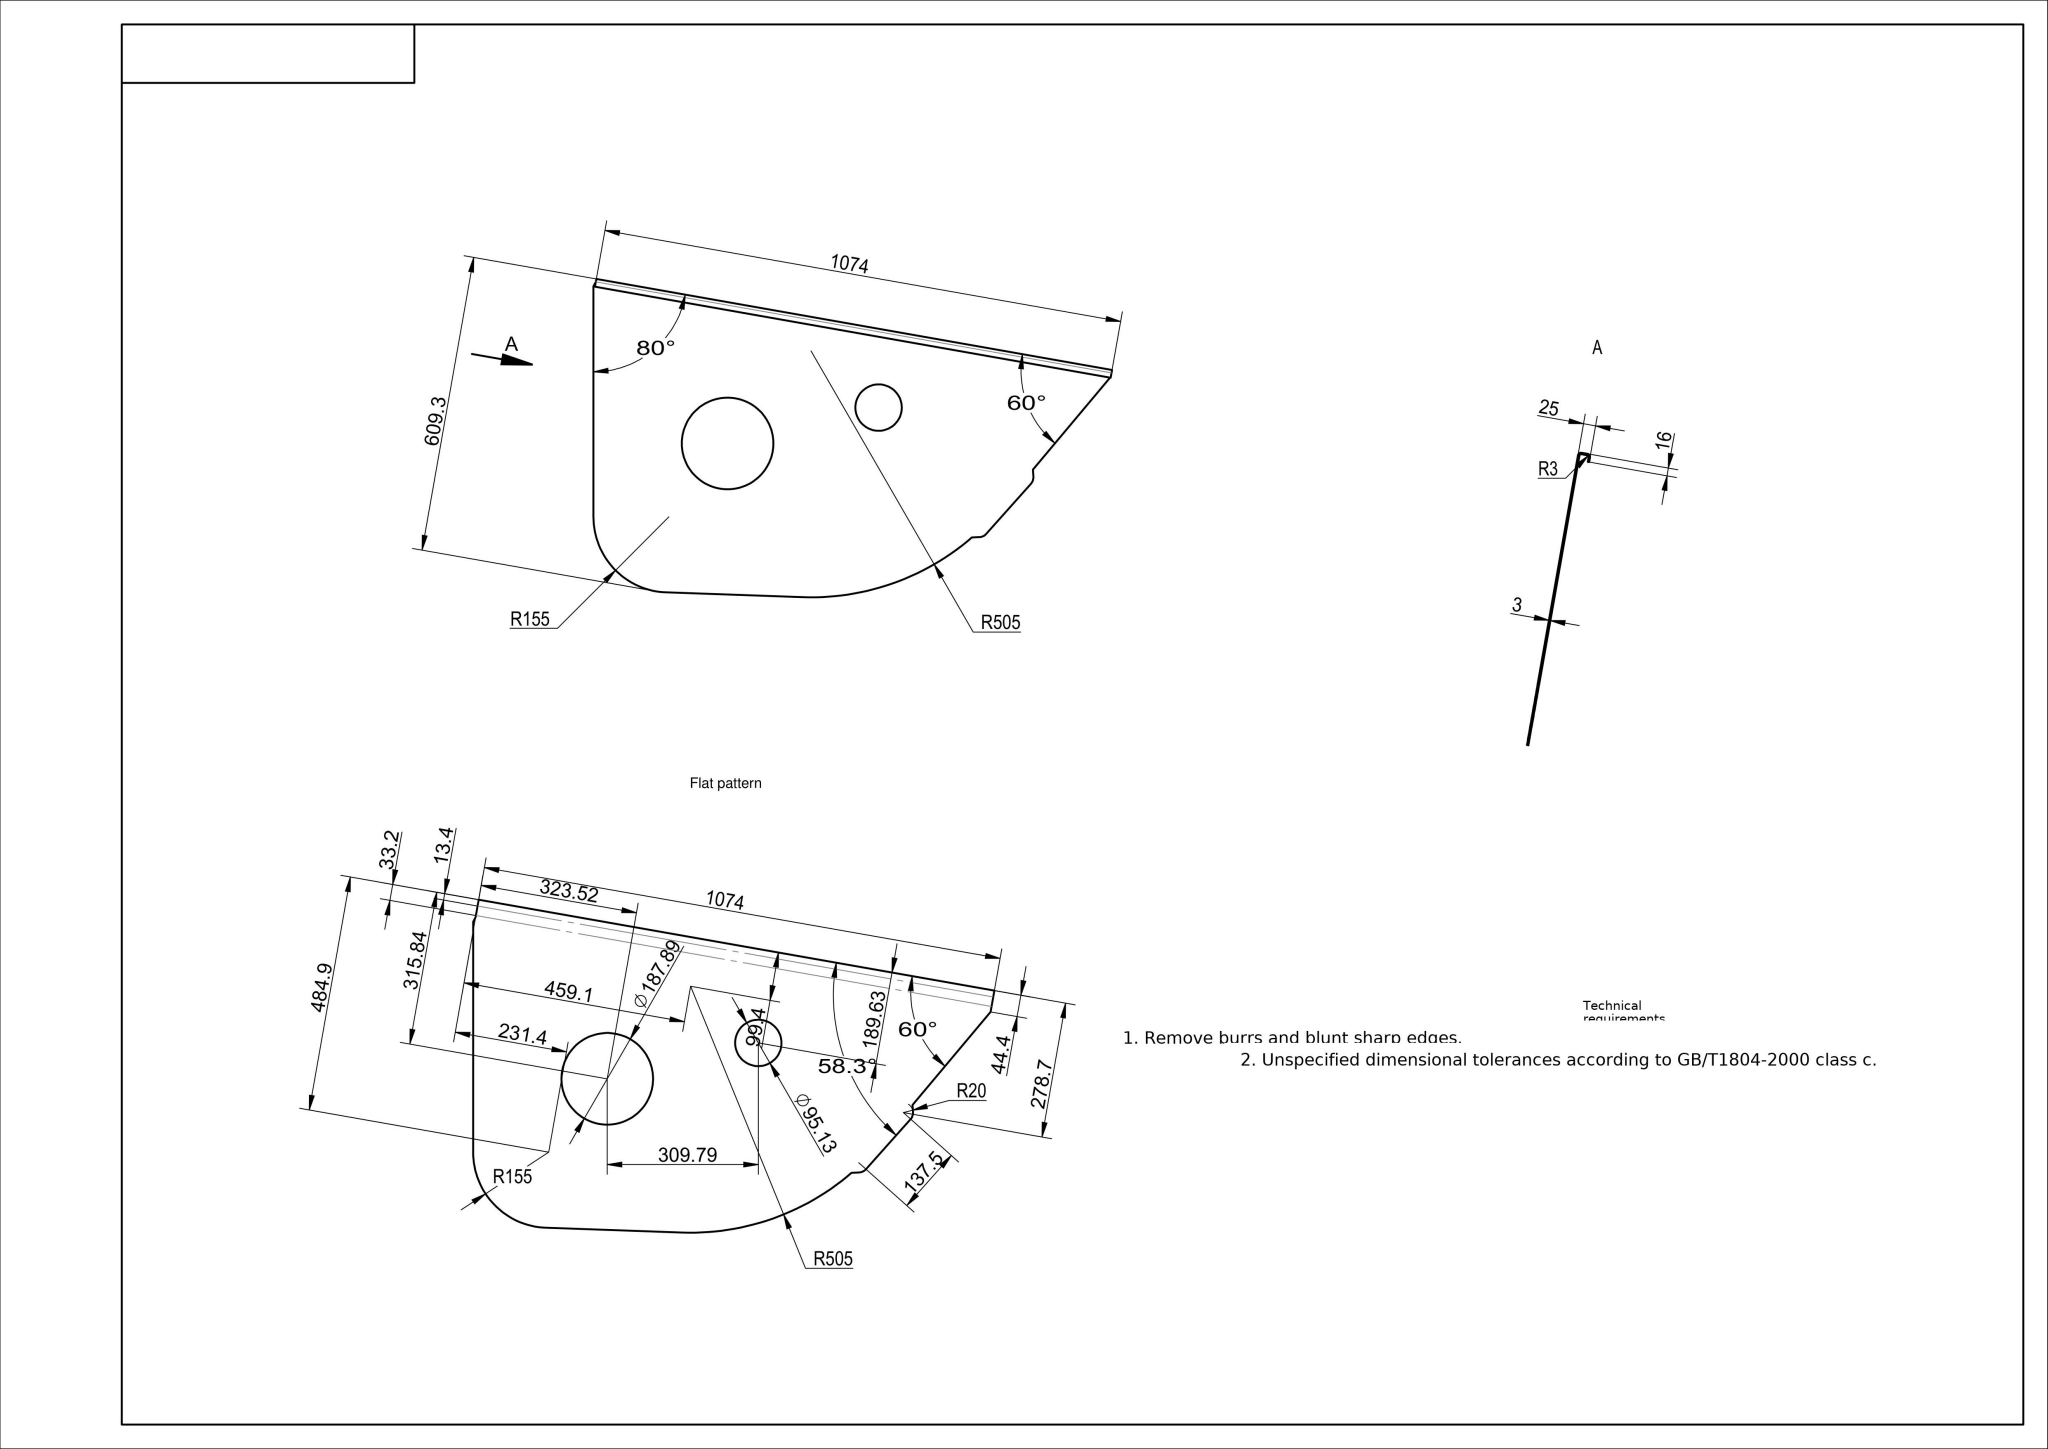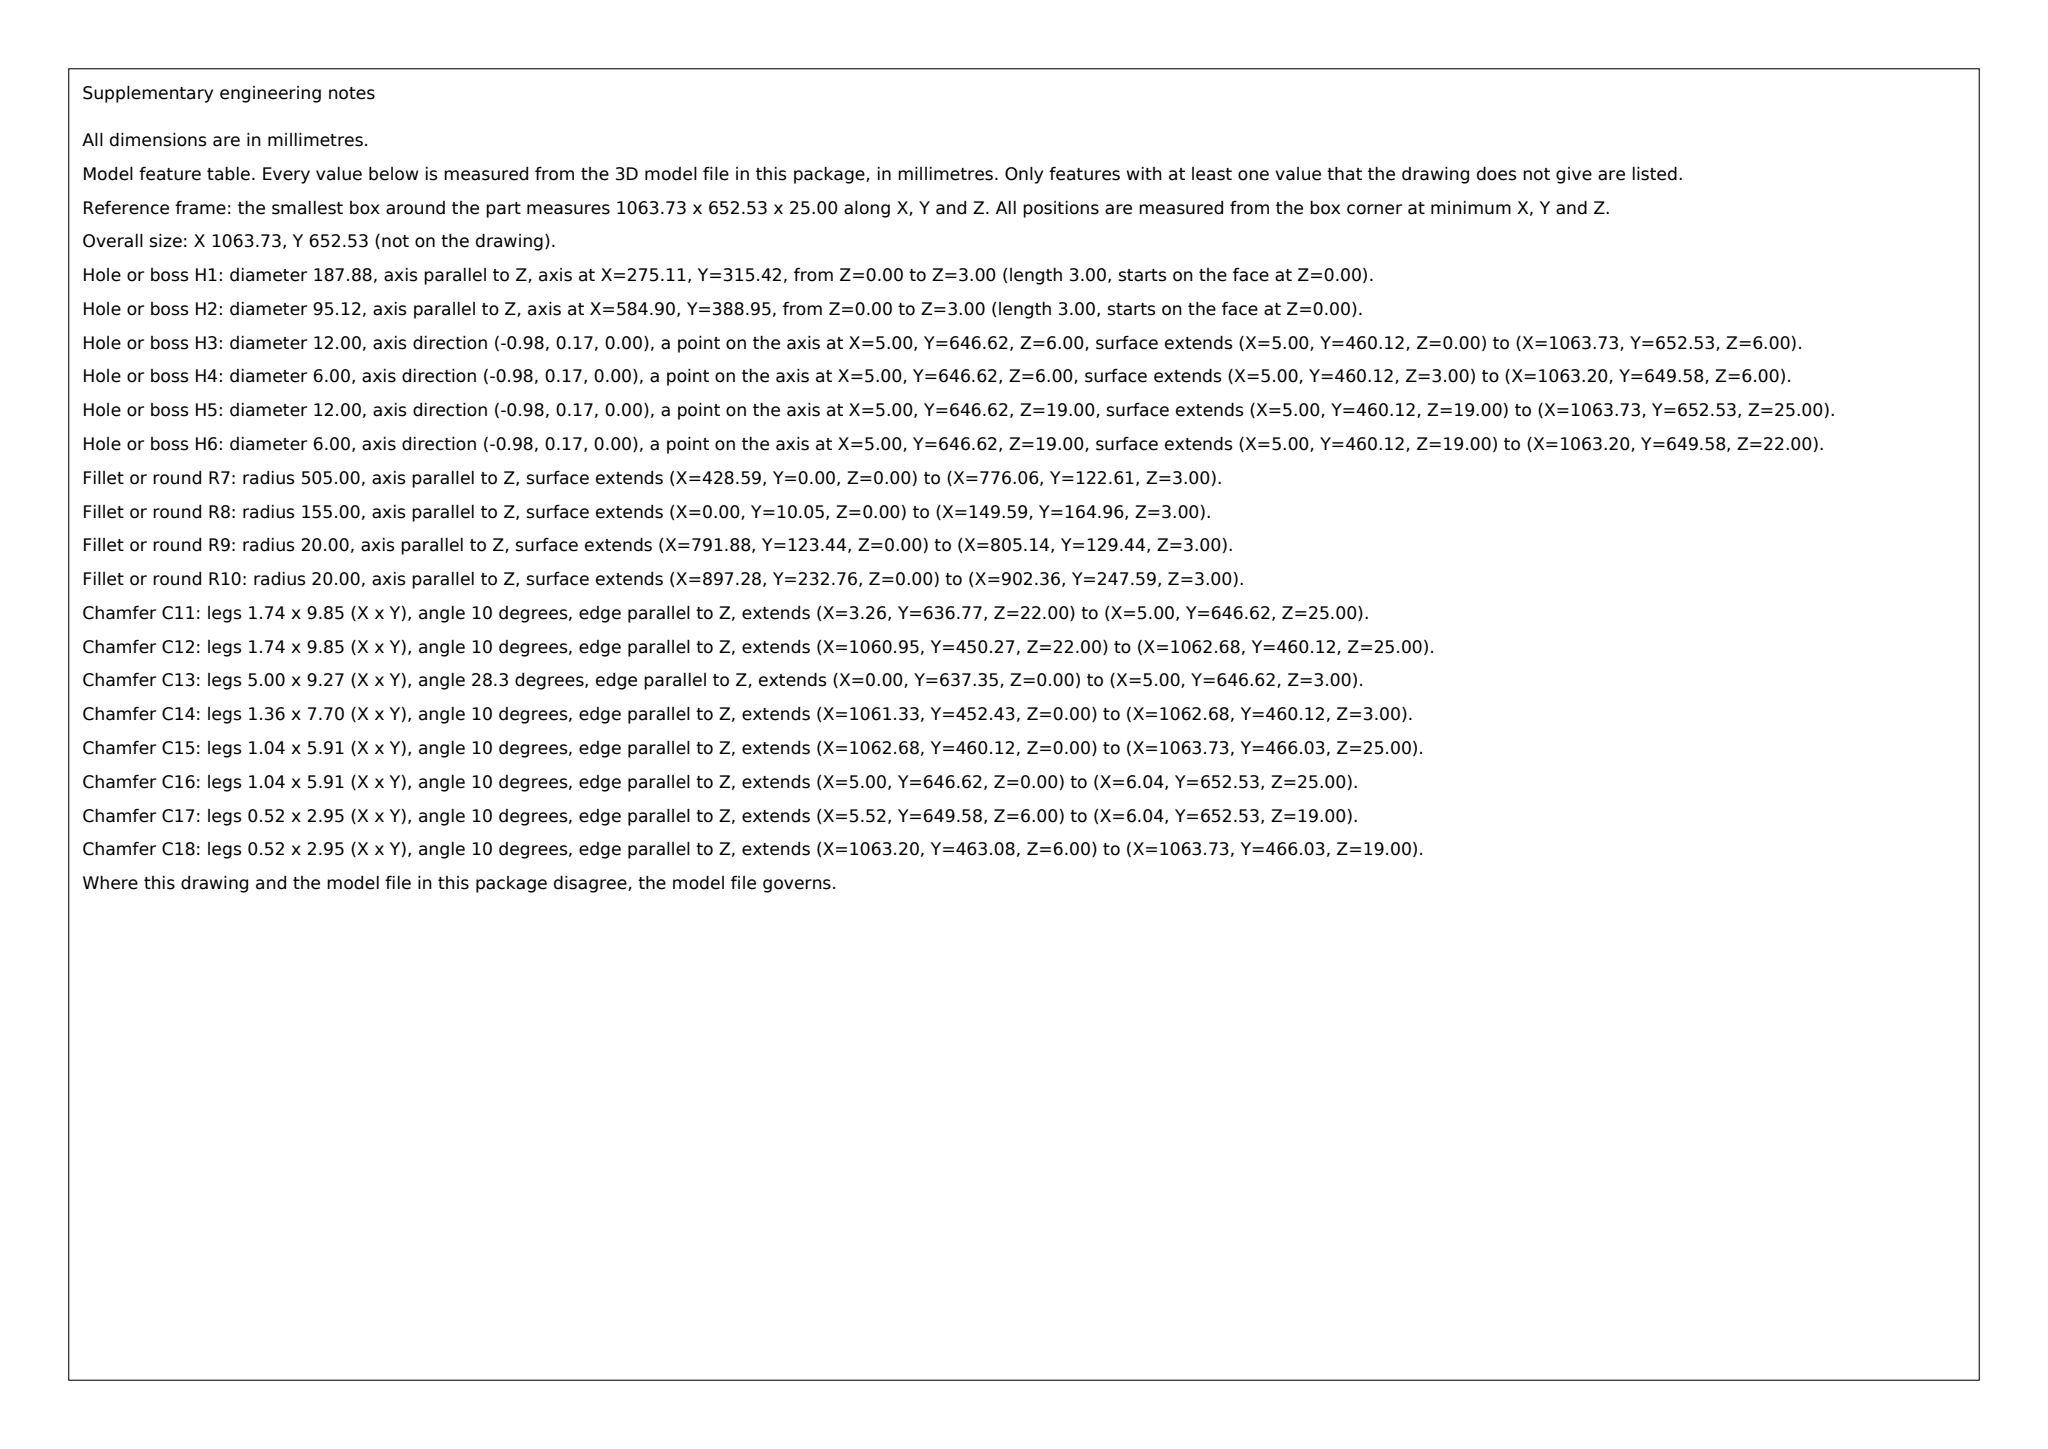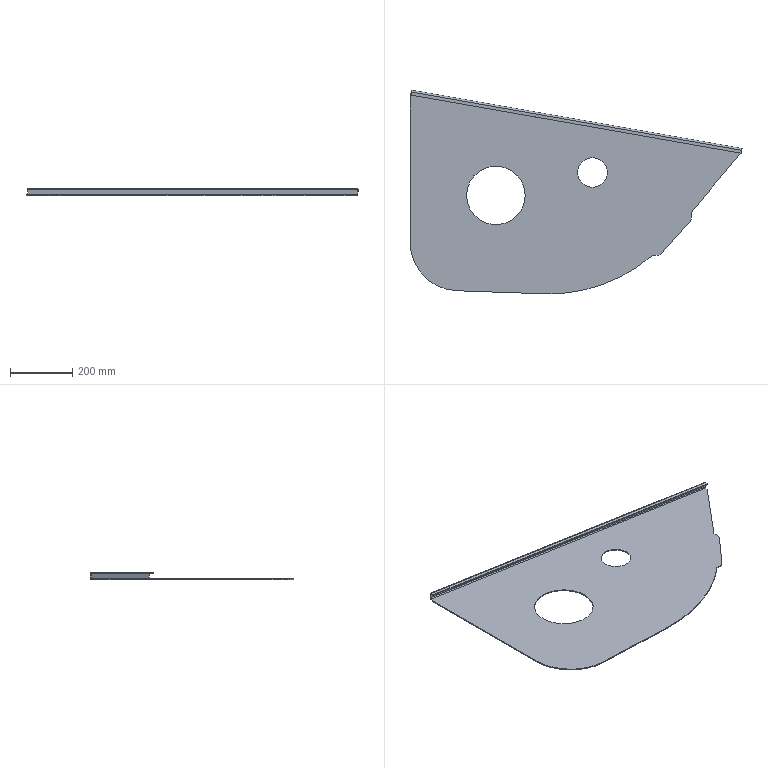Part | SolidWorks | mm | 1 solid | 35 faces | box 1063.73 x 652.53 x 25 mm | volume 1481167 mm3 | plane 23 | cylinder 12 | commonest cylinder face diameters 187.889 x2 95.128 x2 40 x2 12 x2 6 x2 1010 x1 310 x1